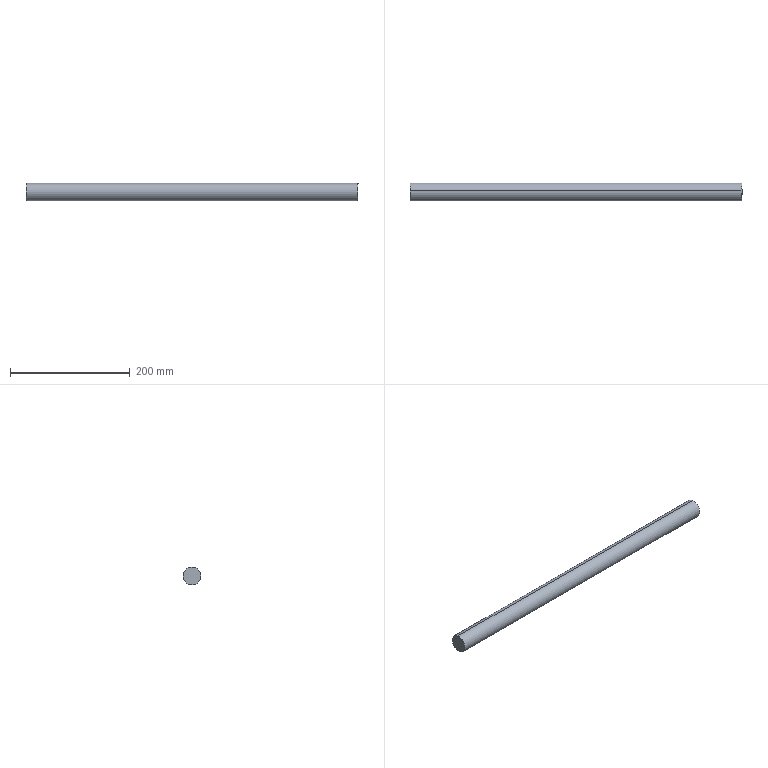Component | SolidWorks | Axis-1 | 1 solid | 4 faces | box 555 x 30 x 30 mm | volume 392306 mm3 | cylinder 2 | plane 2 | commonest cylinder face diameters 30 x2
build123d program:
from build123d import *

# Parameters (mm, degrees)
BOSS_EXTRUDE1_DEPTH      = 10
BOSS_EXTRUDE1_DEPTH_BACK = 545
SKETCH1_R                = 15


with BuildPart() as part:
    # Sketch1 → Boss-Extrude1 (new, two sides: drawn at the far end of the back side and taken through both)
    with BuildSketch(Plane.XY.offset(-BOSS_EXTRUDE1_DEPTH_BACK)):
        Circle(SKETCH1_R)
    extrude(amount=BOSS_EXTRUDE1_DEPTH + BOSS_EXTRUDE1_DEPTH_BACK)


solid = part.part

# Placed as in the assembly
solid = solid.moved(Location((897.268, 164.666, 811.399), (0, 90, 0)))
STEP:
#1=COLOUR_RGB('',0.7922,0.8196,0.9333);
#2=FILL_AREA_STYLE_COLOUR('',#1);
#3=FILL_AREA_STYLE('',(#2));
#4=SURFACE_STYLE_FILL_AREA(#3);
#5=SURFACE_SIDE_STYLE('',(#4));
#6=SURFACE_STYLE_USAGE(.BOTH.,#5);
#7=PRESENTATION_STYLE_ASSIGNMENT((#6));
#8=CARTESIAN_POINT('',(13.869,6.551,32.531));
#9=VERTEX_POINT('',#8);
#10=CARTESIAN_POINT('',(13.869,6.414,31.358));
#11=VERTEX_POINT('',#10);
#12=CARTESIAN_POINT('',(13.869,6.483,31.945));
#13=DIRECTION('',(1.,0.,-0.));
#14=DIRECTION('',(0.,0.1158,0.9933));
#15=AXIS2_PLACEMENT_3D('',#12,#13,#14);
#16=CIRCLE('',#15,0.5906);
#17=EDGE_CURVE('',#9,#11,#16,.T.);
#18=ORIENTED_EDGE('',*,*,#17,.T.);
#19=CARTESIAN_POINT('',(35.719,6.414,31.358));
#20=VERTEX_POINT('',#19);
#21=CARTESIAN_POINT('',(13.869,6.414,31.358));
#22=DIRECTION('',(1.,0.,-0.));
#23=VECTOR('',#22,39.37);
#24=LINE('',#21,#23);
#25=EDGE_CURVE('',#11,#20,#24,.T.);
#26=ORIENTED_EDGE('',*,*,#25,.T.);
#27=CARTESIAN_POINT('',(35.719,6.551,32.531));
#28=VERTEX_POINT('',#27);
#29=CARTESIAN_POINT('',(35.719,6.483,31.945));
#30=DIRECTION('',(1.,0.,-0.));
#31=DIRECTION('',(0.,0.1158,0.9933));
#32=AXIS2_PLACEMENT_3D('',#29,#30,#31);
#33=CIRCLE('',#32,0.5906);
#34=EDGE_CURVE('',#28,#20,#33,.T.);
#35=ORIENTED_EDGE('',*,*,#34,.F.);
#36=CARTESIAN_POINT('',(13.869,6.551,32.531));
#37=DIRECTION('',(1.,0.,-0.));
#38=VECTOR('',#37,39.37);
#39=LINE('',#36,#38);
#40=EDGE_CURVE('',#9,#28,#39,.T.);
#41=ORIENTED_EDGE('',*,*,#40,.F.);
#42=EDGE_LOOP('',(#18,#26,#35,#41));
#43=FACE_OUTER_BOUND('',#42,.T.);
#44=CARTESIAN_POINT('',(13.869,6.483,31.945));
#45=DIRECTION('',(1.,0.,-0.));
#46=DIRECTION('',(0.,0.1158,0.9933));
#47=AXIS2_PLACEMENT_3D('',#44,#45,#46);
#48=CYLINDRICAL_SURFACE('',#47,0.5906);
#49=ADVANCED_FACE('',(#43),#48,.T.);
#50=ORIENTED_EDGE('',*,*,#25,.F.);
#51=CARTESIAN_POINT('',(13.869,6.483,31.945));
#52=DIRECTION('',(1.,0.,-0.));
#53=DIRECTION('',(0.,0.1158,0.9933));
#54=AXIS2_PLACEMENT_3D('',#51,#52,#53);
#55=CIRCLE('',#54,0.5906);
#56=EDGE_CURVE('',#11,#9,#55,.T.);
#57=ORIENTED_EDGE('',*,*,#56,.T.);
#58=ORIENTED_EDGE('',*,*,#40,.T.);
#59=CARTESIAN_POINT('',(35.719,6.483,31.945));
#60=DIRECTION('',(1.,0.,-0.));
#61=DIRECTION('',(0.,0.1158,0.9933));
#62=AXIS2_PLACEMENT_3D('',#59,#60,#61);
#63=CIRCLE('',#62,0.5906);
#64=EDGE_CURVE('',#20,#28,#63,.T.);
#65=ORIENTED_EDGE('',*,*,#64,.F.);
#66=EDGE_LOOP('',(#50,#57,#58,#65));
#67=FACE_OUTER_BOUND('',#66,.T.);
#68=CARTESIAN_POINT('',(13.869,6.483,31.945));
#69=DIRECTION('',(1.,0.,-0.));
#70=DIRECTION('',(0.,0.1158,0.9933));
#71=AXIS2_PLACEMENT_3D('',#68,#69,#70);
#72=CYLINDRICAL_SURFACE('',#71,0.5906);
#73=ADVANCED_FACE('',(#67),#72,.T.);
#74=ORIENTED_EDGE('',*,*,#17,.F.);
#75=ORIENTED_EDGE('',*,*,#56,.F.);
#76=EDGE_LOOP('',(#74,#75));
#77=FACE_OUTER_BOUND('',#76,.T.);
#78=CARTESIAN_POINT('',(13.869,6.483,31.945));
#79=DIRECTION('',(1.,0.,-0.));
#80=DIRECTION('',(0.,0.1158,0.9933));
#81=AXIS2_PLACEMENT_3D('',#78,#79,#80);
#82=PLANE('',#81);
#83=ADVANCED_FACE('',(#77),#82,.F.);
#84=ORIENTED_EDGE('',*,*,#34,.T.);
#85=ORIENTED_EDGE('',*,*,#64,.T.);
#86=EDGE_LOOP('',(#84,#85));
#87=FACE_OUTER_BOUND('',#86,.T.);
#88=CARTESIAN_POINT('',(35.719,6.483,31.945));
#89=DIRECTION('',(1.,0.,-0.));
#90=DIRECTION('',(0.,0.1158,0.9933));
#91=AXIS2_PLACEMENT_3D('',#88,#89,#90);
#92=PLANE('',#91);
#93=ADVANCED_FACE('',(#87),#92,.T.);
#94=CLOSED_SHELL('',(#49,#73,#83,#93));
#95=MANIFOLD_SOLID_BREP('',#94);
#96=STYLED_ITEM('',(#7),#95);
#97=(LENGTH_UNIT()NAMED_UNIT(*)SI_UNIT($,.METRE.));
#98=LENGTH_MEASURE_WITH_UNIT(LENGTH_MEASURE(0.0254),#97);
#99=DIMENSIONAL_EXPONENTS(1.,0.,0.,0.,0.,0.,0.);
#100=(CONVERSION_BASED_UNIT('',#98)LENGTH_UNIT()NAMED_UNIT(#99));
#101=UNCERTAINTY_MEASURE_WITH_UNIT(LENGTH_MEASURE(0.00001),#100,'','');
#102=(NAMED_UNIT(*)PLANE_ANGLE_UNIT()SI_UNIT($,.RADIAN.));
#103=(NAMED_UNIT(*)SI_UNIT($,.STERADIAN.)SOLID_ANGLE_UNIT());
#104=(GEOMETRIC_REPRESENTATION_CONTEXT(3)GLOBAL_UNCERTAINTY_ASSIGNED_CONTEXT((#101))GLOBAL_UNIT_ASSIGNED_CONTEXT((#100,#102,#103))REPRESENTATION_CONTEXT('',''));
#105=MECHANICAL_DESIGN_GEOMETRIC_PRESENTATION_REPRESENTATION('',(#96),#104);
#106=PRESENTATION_LAYER_ASSIGNMENT('','',(#96));
#107=CARTESIAN_POINT('',(0.,0.,0.));
#108=DIRECTION('',(0.,0.,1.));
#109=DIRECTION('',(1.,0.,0.));
#110=AXIS2_PLACEMENT_3D('',#107,#108,#109);
#111=(LENGTH_UNIT()NAMED_UNIT(*)SI_UNIT($,.METRE.));
#112=LENGTH_MEASURE_WITH_UNIT(LENGTH_MEASURE(0.0254),#111);
#113=DIMENSIONAL_EXPONENTS(1.,0.,0.,0.,0.,0.,0.);
#114=(CONVERSION_BASED_UNIT('',#112)LENGTH_UNIT()NAMED_UNIT(#113));
#115=UNCERTAINTY_MEASURE_WITH_UNIT(LENGTH_MEASURE(0.00001),#114,'','');
#116=(NAMED_UNIT(*)PLANE_ANGLE_UNIT()SI_UNIT($,.RADIAN.));
#117=(NAMED_UNIT(*)SI_UNIT($,.STERADIAN.)SOLID_ANGLE_UNIT());
#118=(GEOMETRIC_REPRESENTATION_CONTEXT(3)GLOBAL_UNCERTAINTY_ASSIGNED_CONTEXT((#115))GLOBAL_UNIT_ASSIGNED_CONTEXT((#114,#116,#117))REPRESENTATION_CONTEXT('',''));
#119=ADVANCED_BREP_SHAPE_REPRESENTATION('',(#95,#110),#118);